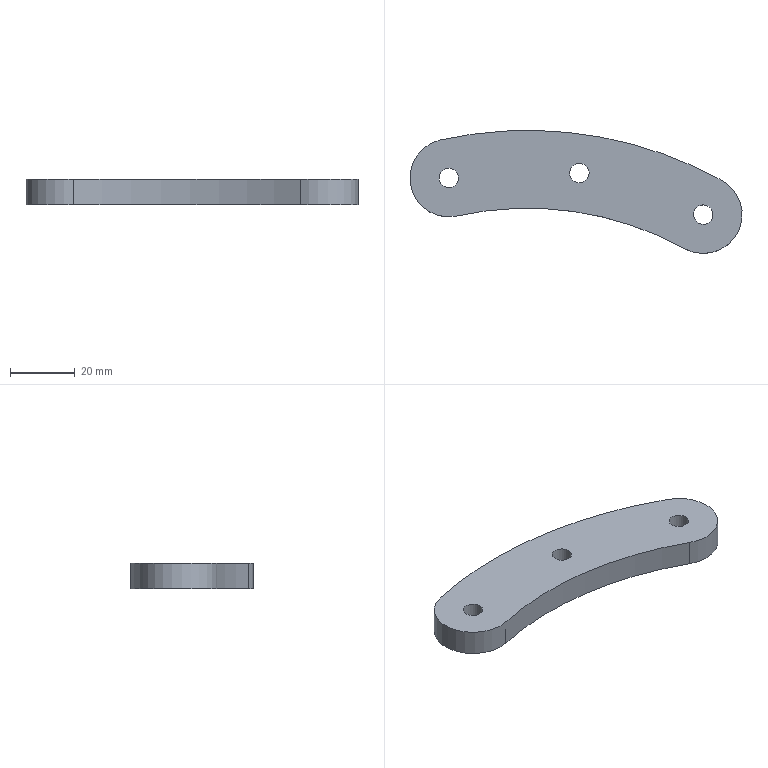Component | NX | 4 | 1 solid | 9 faces | box 102.51 x 37.97 x 8 mm | volume 18508 mm3 | cylinder 7 | plane 2 | commonest cylinder face diameters 6 x3 24 x2 199.98 x1 247.98 x1
STEP:
#1=CARTESIAN_POINT('',(0.,0.,0.));
#2=DIRECTION('',(0.,0.,1.));
#3=DIRECTION('',(1.,0.,0.));
#4=AXIS2_PLACEMENT_3D('',#1,#2,#3);
#5=CARTESIAN_POINT('',(326.775,49.713,-8.));
#6=VERTEX_POINT('',#5);
#7=CARTESIAN_POINT('',(331.992,26.287,-8.));
#8=VERTEX_POINT('',#7);
#9=CARTESIAN_POINT('',(329.383,38.,-8.));
#10=DIRECTION('',(0.,0.,1.));
#11=DIRECTION('',(0.9898,-0.1424,0.));
#12=AXIS2_PLACEMENT_3D('',#9,#10,#11);
#13=CIRCLE('',#12,12.);
#14=CARTESIAN_POINT('',(329.383,38.,0.));
#15=DIRECTION('',(0.,0.,-1.));
#16=DIRECTION('',(-0.9898,0.1424,0.));
#17=AXIS2_PLACEMENT_3D('',#14,#15,#16);
#18=CYLINDRICAL_SURFACE('',#17,12.);
#19=CARTESIAN_POINT('',(9.425,8.));
#20=DIRECTION('',(-1.,0.));
#21=VECTOR('',#20,1.);
#22=LINE('',#19,#21);
#23=(GEOMETRIC_REPRESENTATION_CONTEXT(2)PARAMETRIC_REPRESENTATION_CONTEXT()REPRESENTATION_CONTEXT('',''));
#24=DEFINITIONAL_REPRESENTATION('',(#22),#23);
#25=PCURVE('',#18,#24);
#26=CARTESIAN_POINT('',(341.555,-16.656,-8.));
#27=DIRECTION('',(0.,0.,1.));
#28=DIRECTION('',(0.9898,-0.1424,0.));
#29=AXIS2_PLACEMENT_3D('',#26,#27,#28);
#30=PLANE('',#29);
#31=CARTESIAN_POINT('',(-19.83,52.366));
#32=DIRECTION('',(1.,0.));
#33=AXIS2_PLACEMENT_2D('',#31,#32);
#34=CIRCLE('',#33,12.);
#35=(GEOMETRIC_REPRESENTATION_CONTEXT(2)PARAMETRIC_REPRESENTATION_CONTEXT()REPRESENTATION_CONTEXT('',''));
#36=DEFINITIONAL_REPRESENTATION('',(#34),#35);
#37=PCURVE('',#30,#36);
#38=SURFACE_CURVE('',#13,(#25,#37),.PCURVE_S1.);
#39=EDGE_CURVE('',#6,#8,#38,.T.);
#40=ORIENTED_EDGE('',*,*,#39,.T.);
#41=CARTESIAN_POINT('',(331.992,26.287,0.));
#42=VERTEX_POINT('',#41);
#43=CARTESIAN_POINT('',(331.992,26.287,0.));
#44=DIRECTION('',(0.,0.,-1.));
#45=VECTOR('',#44,1.);
#46=LINE('',#43,#45);
#47=CARTESIAN_POINT('',(4.35,0.));
#48=DIRECTION('',(0.,1.));
#49=VECTOR('',#48,1.);
#50=LINE('',#47,#49);
#51=(GEOMETRIC_REPRESENTATION_CONTEXT(2)PARAMETRIC_REPRESENTATION_CONTEXT()REPRESENTATION_CONTEXT('',''));
#52=DEFINITIONAL_REPRESENTATION('',(#50),#51);
#53=PCURVE('',#18,#52);
#54=CARTESIAN_POINT('',(353.727,-71.312,0.));
#55=DIRECTION('',(0.,0.,-1.));
#56=DIRECTION('',(-0.9898,0.1424,0.));
#57=AXIS2_PLACEMENT_3D('',#54,#55,#56);
#58=CYLINDRICAL_SURFACE('',#57,99.99);
#59=CARTESIAN_POINT('',(1.209,0.));
#60=DIRECTION('',(0.,1.));
#61=VECTOR('',#60,1.);
#62=LINE('',#59,#61);
#63=(GEOMETRIC_REPRESENTATION_CONTEXT(2)PARAMETRIC_REPRESENTATION_CONTEXT()REPRESENTATION_CONTEXT('',''));
#64=DEFINITIONAL_REPRESENTATION('',(#62),#63);
#65=PCURVE('',#58,#64);
#66=SURFACE_CURVE('',#46,(#53,#65),.PCURVE_S1.);
#67=EDGE_CURVE('',#42,#8,#66,.T.);
#68=ORIENTED_EDGE('',*,*,#67,.F.);
#69=CARTESIAN_POINT('',(326.775,49.713,0.));
#70=VERTEX_POINT('',#69);
#71=CARTESIAN_POINT('',(329.383,38.,0.));
#72=DIRECTION('',(0.,0.,1.));
#73=DIRECTION('',(0.9898,-0.1424,0.));
#74=AXIS2_PLACEMENT_3D('',#71,#72,#73);
#75=CIRCLE('',#74,12.);
#76=CARTESIAN_POINT('',(9.425,0.));
#77=DIRECTION('',(-1.,0.));
#78=VECTOR('',#77,1.);
#79=LINE('',#76,#78);
#80=(GEOMETRIC_REPRESENTATION_CONTEXT(2)PARAMETRIC_REPRESENTATION_CONTEXT()REPRESENTATION_CONTEXT('',''));
#81=DEFINITIONAL_REPRESENTATION('',(#79),#80);
#82=PCURVE('',#18,#81);
#83=CARTESIAN_POINT('',(341.555,-16.656,0.));
#84=DIRECTION('',(0.,0.,1.));
#85=DIRECTION('',(0.9898,-0.1424,0.));
#86=AXIS2_PLACEMENT_3D('',#83,#84,#85);
#87=PLANE('',#86);
#88=CARTESIAN_POINT('',(-19.83,52.366));
#89=DIRECTION('',(1.,0.));
#90=AXIS2_PLACEMENT_2D('',#88,#89);
#91=CIRCLE('',#90,12.);
#92=(GEOMETRIC_REPRESENTATION_CONTEXT(2)PARAMETRIC_REPRESENTATION_CONTEXT()REPRESENTATION_CONTEXT('',''));
#93=DEFINITIONAL_REPRESENTATION('',(#91),#92);
#94=PCURVE('',#87,#93);
#95=SURFACE_CURVE('',#75,(#82,#94),.PCURVE_S1.);
#96=EDGE_CURVE('',#70,#42,#95,.T.);
#97=ORIENTED_EDGE('',*,*,#96,.F.);
#98=CARTESIAN_POINT('',(326.775,49.713,0.));
#99=DIRECTION('',(0.,0.,-1.));
#100=VECTOR('',#99,1.);
#101=LINE('',#98,#100);
#102=CARTESIAN_POINT('',(7.492,0.));
#103=DIRECTION('',(0.,1.));
#104=VECTOR('',#103,1.);
#105=LINE('',#102,#104);
#106=(GEOMETRIC_REPRESENTATION_CONTEXT(2)PARAMETRIC_REPRESENTATION_CONTEXT()REPRESENTATION_CONTEXT('',''));
#107=DEFINITIONAL_REPRESENTATION('',(#105),#106);
#108=PCURVE('',#18,#107);
#109=CARTESIAN_POINT('',(353.727,-71.312,0.));
#110=DIRECTION('',(0.,0.,-1.));
#111=DIRECTION('',(-0.9898,0.1424,0.));
#112=AXIS2_PLACEMENT_3D('',#109,#110,#111);
#113=CYLINDRICAL_SURFACE('',#112,123.99);
#114=CARTESIAN_POINT('',(1.209,0.));
#115=DIRECTION('',(0.,1.));
#116=VECTOR('',#115,1.);
#117=LINE('',#114,#116);
#118=(GEOMETRIC_REPRESENTATION_CONTEXT(2)PARAMETRIC_REPRESENTATION_CONTEXT()REPRESENTATION_CONTEXT('',''));
#119=DEFINITIONAL_REPRESENTATION('',(#117),#118);
#120=PCURVE('',#113,#119);
#121=SURFACE_CURVE('',#101,(#108,#120),.PCURVE_S1.);
#122=EDGE_CURVE('',#70,#6,#121,.T.);
#123=ORIENTED_EDGE('',*,*,#122,.T.);
#124=EDGE_LOOP('',(#40,#68,#97,#123));
#125=FACE_BOUND('',#124,.T.);
#126=ADVANCED_FACE('',(#125),#18,.T.);
#127=ORIENTED_EDGE('',*,*,#67,.F.);
#128=CARTESIAN_POINT('',(402.091,16.203,0.));
#129=VERTEX_POINT('',#128);
#130=CARTESIAN_POINT('',(353.727,-71.312,0.));
#131=DIRECTION('',(0.,0.,-1.));
#132=DIRECTION('',(0.9898,-0.1424,0.));
#133=AXIS2_PLACEMENT_3D('',#130,#131,#132);
#134=CIRCLE('',#133,99.99);
#135=CARTESIAN_POINT('',(-3.142,0.));
#136=DIRECTION('',(1.,0.));
#137=VECTOR('',#136,1.);
#138=LINE('',#135,#137);
#139=(GEOMETRIC_REPRESENTATION_CONTEXT(2)PARAMETRIC_REPRESENTATION_CONTEXT()REPRESENTATION_CONTEXT('',''));
#140=DEFINITIONAL_REPRESENTATION('',(#138),#139);
#141=PCURVE('',#58,#140);
#142=CARTESIAN_POINT('',(119.82,-52.366));
#143=CARTESIAN_POINT('',(119.82,-225.554));
#144=CARTESIAN_POINT('',(-30.165,-138.96));
#145=CARTESIAN_POINT('',(-180.15,-52.366));
#146=CARTESIAN_POINT('',(-30.165,34.228));
#147=CARTESIAN_POINT('',(119.82,120.822));
#148=CARTESIAN_POINT('',(119.82,-52.366));
#149=(BOUNDED_CURVE()B_SPLINE_CURVE(2,(#142,#143,#144,#145,#146,#147,#148),.UNSPECIFIED.,.T.,.F.)B_SPLINE_CURVE_WITH_KNOTS((1,2,2,2,2,1),(-2.094,0.,2.094,4.189,6.283,8.378),.UNSPECIFIED.)CURVE()GEOMETRIC_REPRESENTATION_ITEM()RATIONAL_B_SPLINE_CURVE((1.,0.5,1.,0.5,1.,0.5,1.))REPRESENTATION_ITEM(''));
#150=(GEOMETRIC_REPRESENTATION_CONTEXT(2)PARAMETRIC_REPRESENTATION_CONTEXT()REPRESENTATION_CONTEXT('',''));
#151=DEFINITIONAL_REPRESENTATION('',(#149),#150);
#152=PCURVE('',#87,#151);
#153=SURFACE_CURVE('',#134,(#141,#152),.PCURVE_S1.);
#154=EDGE_CURVE('',#42,#129,#153,.T.);
#155=ORIENTED_EDGE('',*,*,#154,.T.);
#156=CARTESIAN_POINT('',(402.091,16.203,-8.));
#157=VERTEX_POINT('',#156);
#158=CARTESIAN_POINT('',(402.091,16.203,0.));
#159=DIRECTION('',(0.,0.,-1.));
#160=VECTOR('',#159,1.);
#161=LINE('',#158,#160);
#162=CARTESIAN_POINT('',(1.933,0.));
#163=DIRECTION('',(0.,1.));
#164=VECTOR('',#163,1.);
#165=LINE('',#162,#164);
#166=(GEOMETRIC_REPRESENTATION_CONTEXT(2)PARAMETRIC_REPRESENTATION_CONTEXT()REPRESENTATION_CONTEXT('',''));
#167=DEFINITIONAL_REPRESENTATION('',(#165),#166);
#168=PCURVE('',#58,#167);
#169=CARTESIAN_POINT('',(407.895,26.706,0.));
#170=DIRECTION('',(0.,0.,-1.));
#171=DIRECTION('',(-0.9898,0.1424,0.));
#172=AXIS2_PLACEMENT_3D('',#169,#170,#171);
#173=CYLINDRICAL_SURFACE('',#172,12.);
#174=CARTESIAN_POINT('',(5.074,0.));
#175=DIRECTION('',(0.,1.));
#176=VECTOR('',#175,1.);
#177=LINE('',#174,#176);
#178=(GEOMETRIC_REPRESENTATION_CONTEXT(2)PARAMETRIC_REPRESENTATION_CONTEXT()REPRESENTATION_CONTEXT('',''));
#179=DEFINITIONAL_REPRESENTATION('',(#177),#178);
#180=PCURVE('',#173,#179);
#181=SURFACE_CURVE('',#161,(#168,#180),.PCURVE_S1.);
#182=EDGE_CURVE('',#129,#157,#181,.T.);
#183=ORIENTED_EDGE('',*,*,#182,.T.);
#184=CARTESIAN_POINT('',(353.727,-71.312,-8.));
#185=DIRECTION('',(0.,0.,-1.));
#186=DIRECTION('',(0.9898,-0.1424,0.));
#187=AXIS2_PLACEMENT_3D('',#184,#185,#186);
#188=CIRCLE('',#187,99.99);
#189=CARTESIAN_POINT('',(-3.142,8.));
#190=DIRECTION('',(1.,0.));
#191=VECTOR('',#190,1.);
#192=LINE('',#189,#191);
#193=(GEOMETRIC_REPRESENTATION_CONTEXT(2)PARAMETRIC_REPRESENTATION_CONTEXT()REPRESENTATION_CONTEXT('',''));
#194=DEFINITIONAL_REPRESENTATION('',(#192),#193);
#195=PCURVE('',#58,#194);
#196=CARTESIAN_POINT('',(119.82,-52.366));
#197=CARTESIAN_POINT('',(119.82,-225.554));
#198=CARTESIAN_POINT('',(-30.165,-138.96));
#199=CARTESIAN_POINT('',(-180.15,-52.366));
#200=CARTESIAN_POINT('',(-30.165,34.228));
#201=CARTESIAN_POINT('',(119.82,120.822));
#202=CARTESIAN_POINT('',(119.82,-52.366));
#203=(BOUNDED_CURVE()B_SPLINE_CURVE(2,(#196,#197,#198,#199,#200,#201,#202),.UNSPECIFIED.,.T.,.F.)B_SPLINE_CURVE_WITH_KNOTS((1,2,2,2,2,1),(-2.094,0.,2.094,4.189,6.283,8.378),.UNSPECIFIED.)CURVE()GEOMETRIC_REPRESENTATION_ITEM()RATIONAL_B_SPLINE_CURVE((1.,0.5,1.,0.5,1.,0.5,1.))REPRESENTATION_ITEM(''));
#204=(GEOMETRIC_REPRESENTATION_CONTEXT(2)PARAMETRIC_REPRESENTATION_CONTEXT()REPRESENTATION_CONTEXT('',''));
#205=DEFINITIONAL_REPRESENTATION('',(#203),#204);
#206=PCURVE('',#30,#205);
#207=SURFACE_CURVE('',#188,(#195,#206),.PCURVE_S1.);
#208=EDGE_CURVE('',#8,#157,#207,.T.);
#209=ORIENTED_EDGE('',*,*,#208,.F.);
#210=EDGE_LOOP('',(#127,#155,#183,#209));
#211=FACE_BOUND('',#210,.F.);
#212=ADVANCED_FACE('',(#211),#58,.F.);
#213=CARTESIAN_POINT('',(413.7,37.209,-8.));
#214=VERTEX_POINT('',#213);
#215=CARTESIAN_POINT('',(407.895,26.706,-8.));
#216=DIRECTION('',(0.,0.,1.));
#217=DIRECTION('',(0.9898,-0.1424,0.));
#218=AXIS2_PLACEMENT_3D('',#215,#216,#217);
#219=CIRCLE('',#218,12.);
#220=CARTESIAN_POINT('',(9.425,8.));
#221=DIRECTION('',(-1.,0.));
#222=VECTOR('',#221,1.);
#223=LINE('',#220,#222);
#224=(GEOMETRIC_REPRESENTATION_CONTEXT(2)PARAMETRIC_REPRESENTATION_CONTEXT()REPRESENTATION_CONTEXT('',''));
#225=DEFINITIONAL_REPRESENTATION('',(#223),#224);
#226=PCURVE('',#173,#225);
#227=CARTESIAN_POINT('',(59.49,52.366));
#228=DIRECTION('',(1.,0.));
#229=AXIS2_PLACEMENT_2D('',#227,#228);
#230=CIRCLE('',#229,12.);
#231=(GEOMETRIC_REPRESENTATION_CONTEXT(2)PARAMETRIC_REPRESENTATION_CONTEXT()REPRESENTATION_CONTEXT('',''));
#232=DEFINITIONAL_REPRESENTATION('',(#230),#231);
#233=PCURVE('',#30,#232);
#234=SURFACE_CURVE('',#219,(#226,#233),.PCURVE_S1.);
#235=EDGE_CURVE('',#157,#214,#234,.T.);
#236=ORIENTED_EDGE('',*,*,#235,.T.);
#237=CARTESIAN_POINT('',(413.7,37.209,0.));
#238=VERTEX_POINT('',#237);
#239=CARTESIAN_POINT('',(413.7,37.209,0.));
#240=DIRECTION('',(0.,0.,-1.));
#241=VECTOR('',#240,1.);
#242=LINE('',#239,#241);
#243=CARTESIAN_POINT('',(1.933,0.));
#244=DIRECTION('',(0.,1.));
#245=VECTOR('',#244,1.);
#246=LINE('',#243,#245);
#247=(GEOMETRIC_REPRESENTATION_CONTEXT(2)PARAMETRIC_REPRESENTATION_CONTEXT()REPRESENTATION_CONTEXT('',''));
#248=DEFINITIONAL_REPRESENTATION('',(#246),#247);
#249=PCURVE('',#173,#248);
#250=CARTESIAN_POINT('',(1.933,0.));
#251=DIRECTION('',(0.,1.));
#252=VECTOR('',#251,1.);
#253=LINE('',#250,#252);
#254=(GEOMETRIC_REPRESENTATION_CONTEXT(2)PARAMETRIC_REPRESENTATION_CONTEXT()REPRESENTATION_CONTEXT('',''));
#255=DEFINITIONAL_REPRESENTATION('',(#253),#254);
#256=PCURVE('',#113,#255);
#257=SURFACE_CURVE('',#242,(#249,#256),.PCURVE_S1.);
#258=EDGE_CURVE('',#238,#214,#257,.T.);
#259=ORIENTED_EDGE('',*,*,#258,.F.);
#260=CARTESIAN_POINT('',(407.895,26.706,0.));
#261=DIRECTION('',(0.,0.,1.));
#262=DIRECTION('',(0.9898,-0.1424,0.));
#263=AXIS2_PLACEMENT_3D('',#260,#261,#262);
#264=CIRCLE('',#263,12.);
#265=CARTESIAN_POINT('',(9.425,0.));
#266=DIRECTION('',(-1.,0.));
#267=VECTOR('',#266,1.);
#268=LINE('',#265,#267);
#269=(GEOMETRIC_REPRESENTATION_CONTEXT(2)PARAMETRIC_REPRESENTATION_CONTEXT()REPRESENTATION_CONTEXT('',''));
#270=DEFINITIONAL_REPRESENTATION('',(#268),#269);
#271=PCURVE('',#173,#270);
#272=CARTESIAN_POINT('',(59.49,52.366));
#273=DIRECTION('',(1.,0.));
#274=AXIS2_PLACEMENT_2D('',#272,#273);
#275=CIRCLE('',#274,12.);
#276=(GEOMETRIC_REPRESENTATION_CONTEXT(2)PARAMETRIC_REPRESENTATION_CONTEXT()REPRESENTATION_CONTEXT('',''));
#277=DEFINITIONAL_REPRESENTATION('',(#275),#276);
#278=PCURVE('',#87,#277);
#279=SURFACE_CURVE('',#264,(#271,#278),.PCURVE_S1.);
#280=EDGE_CURVE('',#129,#238,#279,.T.);
#281=ORIENTED_EDGE('',*,*,#280,.F.);
#282=ORIENTED_EDGE('',*,*,#182,.T.);
#283=EDGE_LOOP('',(#236,#259,#281,#282));
#284=FACE_BOUND('',#283,.T.);
#285=ADVANCED_FACE('',(#284),#173,.T.);
#286=CARTESIAN_POINT('',(372.642,39.109,0.));
#287=VERTEX_POINT('',#286);
#288=CARTESIAN_POINT('',(369.673,39.537,0.));
#289=DIRECTION('',(0.,0.,1.));
#290=DIRECTION('',(0.9898,-0.1424,0.));
#291=AXIS2_PLACEMENT_3D('',#288,#289,#290);
#292=CIRCLE('',#291,3.);
#293=CARTESIAN_POINT('',(369.673,39.537,0.));
#294=DIRECTION('',(0.,0.,-1.));
#295=DIRECTION('',(-0.9898,0.1424,0.));
#296=AXIS2_PLACEMENT_3D('',#293,#294,#295);
#297=CYLINDRICAL_SURFACE('',#296,3.);
#298=CARTESIAN_POINT('',(9.425,0.));
#299=DIRECTION('',(-1.,0.));
#300=VECTOR('',#299,1.);
#301=LINE('',#298,#300);
#302=(GEOMETRIC_REPRESENTATION_CONTEXT(2)PARAMETRIC_REPRESENTATION_CONTEXT()REPRESENTATION_CONTEXT('',''));
#303=DEFINITIONAL_REPRESENTATION('',(#301),#302);
#304=PCURVE('',#297,#303);
#305=CARTESIAN_POINT('',(19.83,59.624));
#306=DIRECTION('',(1.,-0.));
#307=AXIS2_PLACEMENT_2D('',#305,#306);
#308=CIRCLE('',#307,3.);
#309=(GEOMETRIC_REPRESENTATION_CONTEXT(2)PARAMETRIC_REPRESENTATION_CONTEXT()REPRESENTATION_CONTEXT('',''));
#310=DEFINITIONAL_REPRESENTATION('',(#308),#309);
#311=PCURVE('',#87,#310);
#312=SURFACE_CURVE('',#292,(#304,#311),.PCURVE_S1.);
#313=EDGE_CURVE('',#287,#287,#312,.T.);
#314=ORIENTED_EDGE('',*,*,#313,.F.);
#315=CARTESIAN_POINT('',(372.642,39.109,-8.));
#316=VERTEX_POINT('',#315);
#317=CARTESIAN_POINT('',(372.642,39.109,0.));
#318=CARTESIAN_POINT('',(372.642,39.109,-8.));
#319=B_SPLINE_CURVE_WITH_KNOTS('',1,(#317,#318),.UNSPECIFIED.,.F.,.F.,(2,2),(0.,8.),.PIECEWISE_BEZIER_KNOTS.);
#320=CARTESIAN_POINT('',(9.425,0.));
#321=DIRECTION('',(0.,1.));
#322=VECTOR('',#321,1.);
#323=LINE('',#320,#322);
#324=(GEOMETRIC_REPRESENTATION_CONTEXT(2)PARAMETRIC_REPRESENTATION_CONTEXT()REPRESENTATION_CONTEXT('',''));
#325=DEFINITIONAL_REPRESENTATION('',(#323),#324);
#326=PCURVE('',#297,#325);
#327=CARTESIAN_POINT('',(3.142,0.));
#328=DIRECTION('',(0.,1.));
#329=VECTOR('',#328,1.);
#330=LINE('',#327,#329);
#331=(GEOMETRIC_REPRESENTATION_CONTEXT(2)PARAMETRIC_REPRESENTATION_CONTEXT()REPRESENTATION_CONTEXT('',''));
#332=DEFINITIONAL_REPRESENTATION('',(#330),#331);
#333=PCURVE('',#297,#332);
#334=SEAM_CURVE('',#319,(#326,#333),.PCURVE_S1.);
#335=EDGE_CURVE('',#287,#316,#334,.T.);
#336=ORIENTED_EDGE('',*,*,#335,.T.);
#337=CARTESIAN_POINT('',(369.673,39.537,-8.));
#338=DIRECTION('',(0.,0.,1.));
#339=DIRECTION('',(0.9898,-0.1424,0.));
#340=AXIS2_PLACEMENT_3D('',#337,#338,#339);
#341=CIRCLE('',#340,3.);
#342=CARTESIAN_POINT('',(9.425,8.));
#343=DIRECTION('',(-1.,0.));
#344=VECTOR('',#343,1.);
#345=LINE('',#342,#344);
#346=(GEOMETRIC_REPRESENTATION_CONTEXT(2)PARAMETRIC_REPRESENTATION_CONTEXT()REPRESENTATION_CONTEXT('',''));
#347=DEFINITIONAL_REPRESENTATION('',(#345),#346);
#348=PCURVE('',#297,#347);
#349=CARTESIAN_POINT('',(19.83,59.624));
#350=DIRECTION('',(1.,-0.));
#351=AXIS2_PLACEMENT_2D('',#349,#350);
#352=CIRCLE('',#351,3.);
#353=(GEOMETRIC_REPRESENTATION_CONTEXT(2)PARAMETRIC_REPRESENTATION_CONTEXT()REPRESENTATION_CONTEXT('',''));
#354=DEFINITIONAL_REPRESENTATION('',(#352),#353);
#355=PCURVE('',#30,#354);
#356=SURFACE_CURVE('',#341,(#348,#355),.PCURVE_S1.);
#357=EDGE_CURVE('',#316,#316,#356,.T.);
#358=ORIENTED_EDGE('',*,*,#357,.T.);
#359=ORIENTED_EDGE('',*,*,#335,.F.);
#360=EDGE_LOOP('',(#314,#336,#358,#359));
#361=FACE_BOUND('',#360,.F.);
#362=ADVANCED_FACE('',(#361),#297,.F.);
#363=CARTESIAN_POINT('',(332.353,37.573,0.));
#364=VERTEX_POINT('',#363);
#365=CARTESIAN_POINT('',(329.383,38.,0.));
#366=DIRECTION('',(0.,0.,1.));
#367=DIRECTION('',(0.9898,-0.1424,0.));
#368=AXIS2_PLACEMENT_3D('',#365,#366,#367);
#369=CIRCLE('',#368,3.);
#370=CARTESIAN_POINT('',(329.383,38.,0.));
#371=DIRECTION('',(0.,0.,-1.));
#372=DIRECTION('',(-0.9898,0.1424,0.));
#373=AXIS2_PLACEMENT_3D('',#370,#371,#372);
#374=CYLINDRICAL_SURFACE('',#373,3.);
#375=CARTESIAN_POINT('',(9.425,0.));
#376=DIRECTION('',(-1.,0.));
#377=VECTOR('',#376,1.);
#378=LINE('',#375,#377);
#379=(GEOMETRIC_REPRESENTATION_CONTEXT(2)PARAMETRIC_REPRESENTATION_CONTEXT()REPRESENTATION_CONTEXT('',''));
#380=DEFINITIONAL_REPRESENTATION('',(#378),#379);
#381=PCURVE('',#374,#380);
#382=CARTESIAN_POINT('',(-19.83,52.366));
#383=DIRECTION('',(1.,-0.));
#384=AXIS2_PLACEMENT_2D('',#382,#383);
#385=CIRCLE('',#384,3.);
#386=(GEOMETRIC_REPRESENTATION_CONTEXT(2)PARAMETRIC_REPRESENTATION_CONTEXT()REPRESENTATION_CONTEXT('',''));
#387=DEFINITIONAL_REPRESENTATION('',(#385),#386);
#388=PCURVE('',#87,#387);
#389=SURFACE_CURVE('',#369,(#381,#388),.PCURVE_S1.);
#390=EDGE_CURVE('',#364,#364,#389,.T.);
#391=ORIENTED_EDGE('',*,*,#390,.F.);
#392=CARTESIAN_POINT('',(332.353,37.573,-8.));
#393=VERTEX_POINT('',#392);
#394=CARTESIAN_POINT('',(332.353,37.573,0.));
#395=CARTESIAN_POINT('',(332.353,37.573,-8.));
#396=B_SPLINE_CURVE_WITH_KNOTS('',1,(#394,#395),.UNSPECIFIED.,.F.,.F.,(2,2),(0.,8.),.PIECEWISE_BEZIER_KNOTS.);
#397=CARTESIAN_POINT('',(9.425,0.));
#398=DIRECTION('',(0.,1.));
#399=VECTOR('',#398,1.);
#400=LINE('',#397,#399);
#401=(GEOMETRIC_REPRESENTATION_CONTEXT(2)PARAMETRIC_REPRESENTATION_CONTEXT()REPRESENTATION_CONTEXT('',''));
#402=DEFINITIONAL_REPRESENTATION('',(#400),#401);
#403=PCURVE('',#374,#402);
#404=CARTESIAN_POINT('',(3.142,0.));
#405=DIRECTION('',(0.,1.));
#406=VECTOR('',#405,1.);
#407=LINE('',#404,#406);
#408=(GEOMETRIC_REPRESENTATION_CONTEXT(2)PARAMETRIC_REPRESENTATION_CONTEXT()REPRESENTATION_CONTEXT('',''));
#409=DEFINITIONAL_REPRESENTATION('',(#407),#408);
#410=PCURVE('',#374,#409);
#411=SEAM_CURVE('',#396,(#403,#410),.PCURVE_S1.);
#412=EDGE_CURVE('',#364,#393,#411,.T.);
#413=ORIENTED_EDGE('',*,*,#412,.T.);
#414=CARTESIAN_POINT('',(329.383,38.,-8.));
#415=DIRECTION('',(0.,0.,1.));
#416=DIRECTION('',(0.9898,-0.1424,0.));
#417=AXIS2_PLACEMENT_3D('',#414,#415,#416);
#418=CIRCLE('',#417,3.);
#419=CARTESIAN_POINT('',(9.425,8.));
#420=DIRECTION('',(-1.,0.));
#421=VECTOR('',#420,1.);
#422=LINE('',#419,#421);
#423=(GEOMETRIC_REPRESENTATION_CONTEXT(2)PARAMETRIC_REPRESENTATION_CONTEXT()REPRESENTATION_CONTEXT('',''));
#424=DEFINITIONAL_REPRESENTATION('',(#422),#423);
#425=PCURVE('',#374,#424);
#426=CARTESIAN_POINT('',(-19.83,52.366));
#427=DIRECTION('',(1.,-0.));
#428=AXIS2_PLACEMENT_2D('',#426,#427);
#429=CIRCLE('',#428,3.);
#430=(GEOMETRIC_REPRESENTATION_CONTEXT(2)PARAMETRIC_REPRESENTATION_CONTEXT()REPRESENTATION_CONTEXT('',''));
#431=DEFINITIONAL_REPRESENTATION('',(#429),#430);
#432=PCURVE('',#30,#431);
#433=SURFACE_CURVE('',#418,(#425,#432),.PCURVE_S1.);
#434=EDGE_CURVE('',#393,#393,#433,.T.);
#435=ORIENTED_EDGE('',*,*,#434,.T.);
#436=ORIENTED_EDGE('',*,*,#412,.F.);
#437=EDGE_LOOP('',(#391,#413,#435,#436));
#438=FACE_BOUND('',#437,.F.);
#439=ADVANCED_FACE('',(#438),#374,.F.);
#440=CARTESIAN_POINT('',(353.727,-71.312,-8.));
#441=DIRECTION('',(0.,0.,1.));
#442=DIRECTION('',(0.9898,-0.1424,0.));
#443=AXIS2_PLACEMENT_3D('',#440,#441,#442);
#444=CIRCLE('',#443,123.99);
#445=CARTESIAN_POINT('',(3.142,8.));
#446=DIRECTION('',(-1.,0.));
#447=VECTOR('',#446,1.);
#448=LINE('',#445,#447);
#449=(GEOMETRIC_REPRESENTATION_CONTEXT(2)PARAMETRIC_REPRESENTATION_CONTEXT()REPRESENTATION_CONTEXT('',''));
#450=DEFINITIONAL_REPRESENTATION('',(#448),#449);
#451=PCURVE('',#113,#450);
#452=CARTESIAN_POINT('',(19.83,-52.366));
#453=DIRECTION('',(1.,0.));
#454=AXIS2_PLACEMENT_2D('',#452,#453);
#455=CIRCLE('',#454,123.99);
#456=(GEOMETRIC_REPRESENTATION_CONTEXT(2)PARAMETRIC_REPRESENTATION_CONTEXT()REPRESENTATION_CONTEXT('',''));
#457=DEFINITIONAL_REPRESENTATION('',(#455),#456);
#458=PCURVE('',#30,#457);
#459=SURFACE_CURVE('',#444,(#451,#458),.PCURVE_S1.);
#460=EDGE_CURVE('',#214,#6,#459,.T.);
#461=ORIENTED_EDGE('',*,*,#460,.T.);
#462=ORIENTED_EDGE('',*,*,#122,.F.);
#463=CARTESIAN_POINT('',(353.727,-71.312,0.));
#464=DIRECTION('',(0.,0.,1.));
#465=DIRECTION('',(0.9898,-0.1424,0.));
#466=AXIS2_PLACEMENT_3D('',#463,#464,#465);
#467=CIRCLE('',#466,123.99);
#468=CARTESIAN_POINT('',(3.142,0.));
#469=DIRECTION('',(-1.,0.));
#470=VECTOR('',#469,1.);
#471=LINE('',#468,#470);
#472=(GEOMETRIC_REPRESENTATION_CONTEXT(2)PARAMETRIC_REPRESENTATION_CONTEXT()REPRESENTATION_CONTEXT('',''));
#473=DEFINITIONAL_REPRESENTATION('',(#471),#472);
#474=PCURVE('',#113,#473);
#475=CARTESIAN_POINT('',(19.83,-52.366));
#476=DIRECTION('',(1.,0.));
#477=AXIS2_PLACEMENT_2D('',#475,#476);
#478=CIRCLE('',#477,123.99);
#479=(GEOMETRIC_REPRESENTATION_CONTEXT(2)PARAMETRIC_REPRESENTATION_CONTEXT()REPRESENTATION_CONTEXT('',''));
#480=DEFINITIONAL_REPRESENTATION('',(#478),#479);
#481=PCURVE('',#87,#480);
#482=SURFACE_CURVE('',#467,(#474,#481),.PCURVE_S1.);
#483=EDGE_CURVE('',#238,#70,#482,.T.);
#484=ORIENTED_EDGE('',*,*,#483,.F.);
#485=ORIENTED_EDGE('',*,*,#258,.T.);
#486=EDGE_LOOP('',(#461,#462,#484,#485));
#487=FACE_BOUND('',#486,.T.);
#488=ADVANCED_FACE('',(#487),#113,.T.);
#489=CARTESIAN_POINT('',(410.865,26.279,0.));
#490=VERTEX_POINT('',#489);
#491=CARTESIAN_POINT('',(407.895,26.706,0.));
#492=DIRECTION('',(0.,0.,1.));
#493=DIRECTION('',(0.9898,-0.1424,0.));
#494=AXIS2_PLACEMENT_3D('',#491,#492,#493);
#495=CIRCLE('',#494,3.);
#496=CARTESIAN_POINT('',(407.895,26.706,0.));
#497=DIRECTION('',(0.,0.,-1.));
#498=DIRECTION('',(-0.9898,0.1424,0.));
#499=AXIS2_PLACEMENT_3D('',#496,#497,#498);
#500=CYLINDRICAL_SURFACE('',#499,3.);
#501=CARTESIAN_POINT('',(9.425,0.));
#502=DIRECTION('',(-1.,0.));
#503=VECTOR('',#502,1.);
#504=LINE('',#501,#503);
#505=(GEOMETRIC_REPRESENTATION_CONTEXT(2)PARAMETRIC_REPRESENTATION_CONTEXT()REPRESENTATION_CONTEXT('',''));
#506=DEFINITIONAL_REPRESENTATION('',(#504),#505);
#507=PCURVE('',#500,#506);
#508=CARTESIAN_POINT('',(59.49,52.366));
#509=DIRECTION('',(1.,-0.));
#510=AXIS2_PLACEMENT_2D('',#508,#509);
#511=CIRCLE('',#510,3.);
#512=(GEOMETRIC_REPRESENTATION_CONTEXT(2)PARAMETRIC_REPRESENTATION_CONTEXT()REPRESENTATION_CONTEXT('',''));
#513=DEFINITIONAL_REPRESENTATION('',(#511),#512);
#514=PCURVE('',#87,#513);
#515=SURFACE_CURVE('',#495,(#507,#514),.PCURVE_S1.);
#516=EDGE_CURVE('',#490,#490,#515,.T.);
#517=ORIENTED_EDGE('',*,*,#516,.F.);
#518=CARTESIAN_POINT('',(410.865,26.279,-8.));
#519=VERTEX_POINT('',#518);
#520=CARTESIAN_POINT('',(410.865,26.279,0.));
#521=CARTESIAN_POINT('',(410.865,26.279,-8.));
#522=B_SPLINE_CURVE_WITH_KNOTS('',1,(#520,#521),.UNSPECIFIED.,.F.,.F.,(2,2),(0.,8.),.PIECEWISE_BEZIER_KNOTS.);
#523=CARTESIAN_POINT('',(9.425,0.));
#524=DIRECTION('',(0.,1.));
#525=VECTOR('',#524,1.);
#526=LINE('',#523,#525);
#527=(GEOMETRIC_REPRESENTATION_CONTEXT(2)PARAMETRIC_REPRESENTATION_CONTEXT()REPRESENTATION_CONTEXT('',''));
#528=DEFINITIONAL_REPRESENTATION('',(#526),#527);
#529=PCURVE('',#500,#528);
#530=CARTESIAN_POINT('',(3.142,0.));
#531=DIRECTION('',(0.,1.));
#532=VECTOR('',#531,1.);
#533=LINE('',#530,#532);
#534=(GEOMETRIC_REPRESENTATION_CONTEXT(2)PARAMETRIC_REPRESENTATION_CONTEXT()REPRESENTATION_CONTEXT('',''));
#535=DEFINITIONAL_REPRESENTATION('',(#533),#534);
#536=PCURVE('',#500,#535);
#537=SEAM_CURVE('',#522,(#529,#536),.PCURVE_S1.);
#538=EDGE_CURVE('',#490,#519,#537,.T.);
#539=ORIENTED_EDGE('',*,*,#538,.T.);
#540=CARTESIAN_POINT('',(407.895,26.706,-8.));
#541=DIRECTION('',(0.,0.,1.));
#542=DIRECTION('',(0.9898,-0.1424,0.));
#543=AXIS2_PLACEMENT_3D('',#540,#541,#542);
#544=CIRCLE('',#543,3.);
#545=CARTESIAN_POINT('',(9.425,8.));
#546=DIRECTION('',(-1.,0.));
#547=VECTOR('',#546,1.);
#548=LINE('',#545,#547);
#549=(GEOMETRIC_REPRESENTATION_CONTEXT(2)PARAMETRIC_REPRESENTATION_CONTEXT()REPRESENTATION_CONTEXT('',''));
#550=DEFINITIONAL_REPRESENTATION('',(#548),#549);
#551=PCURVE('',#500,#550);
#552=CARTESIAN_POINT('',(59.49,52.366));
#553=DIRECTION('',(1.,-0.));
#554=AXIS2_PLACEMENT_2D('',#552,#553);
#555=CIRCLE('',#554,3.);
#556=(GEOMETRIC_REPRESENTATION_CONTEXT(2)PARAMETRIC_REPRESENTATION_CONTEXT()REPRESENTATION_CONTEXT('',''));
#557=DEFINITIONAL_REPRESENTATION('',(#555),#556);
#558=PCURVE('',#30,#557);
#559=SURFACE_CURVE('',#544,(#551,#558),.PCURVE_S1.);
#560=EDGE_CURVE('',#519,#519,#559,.T.);
#561=ORIENTED_EDGE('',*,*,#560,.T.);
#562=ORIENTED_EDGE('',*,*,#538,.F.);
#563=EDGE_LOOP('',(#517,#539,#561,#562));
#564=FACE_BOUND('',#563,.F.);
#565=ADVANCED_FACE('',(#564),#500,.F.);
#566=ORIENTED_EDGE('',*,*,#96,.T.);
#567=ORIENTED_EDGE('',*,*,#154,.T.);
#568=ORIENTED_EDGE('',*,*,#280,.T.);
#569=ORIENTED_EDGE('',*,*,#483,.T.);
#570=EDGE_LOOP('',(#566,#567,#568,#569));
#571=FACE_BOUND('',#570,.T.);
#572=ORIENTED_EDGE('',*,*,#390,.F.);
#573=EDGE_LOOP('',(#572));
#574=FACE_BOUND('',#573,.T.);
#575=ORIENTED_EDGE('',*,*,#313,.F.);
#576=EDGE_LOOP('',(#575));
#577=FACE_BOUND('',#576,.T.);
#578=ORIENTED_EDGE('',*,*,#516,.F.);
#579=EDGE_LOOP('',(#578));
#580=FACE_BOUND('',#579,.T.);
#581=ADVANCED_FACE('',(#571,#574,#577,#580),#87,.T.);
#582=ORIENTED_EDGE('',*,*,#39,.F.);
#583=ORIENTED_EDGE('',*,*,#460,.F.);
#584=ORIENTED_EDGE('',*,*,#235,.F.);
#585=ORIENTED_EDGE('',*,*,#208,.F.);
#586=EDGE_LOOP('',(#582,#583,#584,#585));
#587=FACE_BOUND('',#586,.T.);
#588=ORIENTED_EDGE('',*,*,#434,.T.);
#589=EDGE_LOOP('',(#588));
#590=FACE_BOUND('',#589,.T.);
#591=ORIENTED_EDGE('',*,*,#357,.T.);
#592=EDGE_LOOP('',(#591));
#593=FACE_BOUND('',#592,.T.);
#594=ORIENTED_EDGE('',*,*,#560,.T.);
#595=EDGE_LOOP('',(#594));
#596=FACE_BOUND('',#595,.T.);
#597=ADVANCED_FACE('',(#587,#590,#593,#596),#30,.F.);
#598=CLOSED_SHELL('',(#126,#212,#285,#362,#439,#488,#565,#581,#597));
#599=MANIFOLD_SOLID_BREP('',#598);
#600=(LENGTH_UNIT()NAMED_UNIT(*)SI_UNIT(.MILLI.,.METRE.));
#601=UNCERTAINTY_MEASURE_WITH_UNIT(LENGTH_MEASURE(0.000002),#600,'','');
#602=(NAMED_UNIT(*)PLANE_ANGLE_UNIT()SI_UNIT($,.RADIAN.));
#603=(NAMED_UNIT(*)SI_UNIT($,.STERADIAN.)SOLID_ANGLE_UNIT());
#604=(GEOMETRIC_REPRESENTATION_CONTEXT(3)GLOBAL_UNCERTAINTY_ASSIGNED_CONTEXT((#601))GLOBAL_UNIT_ASSIGNED_CONTEXT((#600,#602,#603))REPRESENTATION_CONTEXT('',''));
#605=ADVANCED_BREP_SHAPE_REPRESENTATION('',(#4,#599),#604);